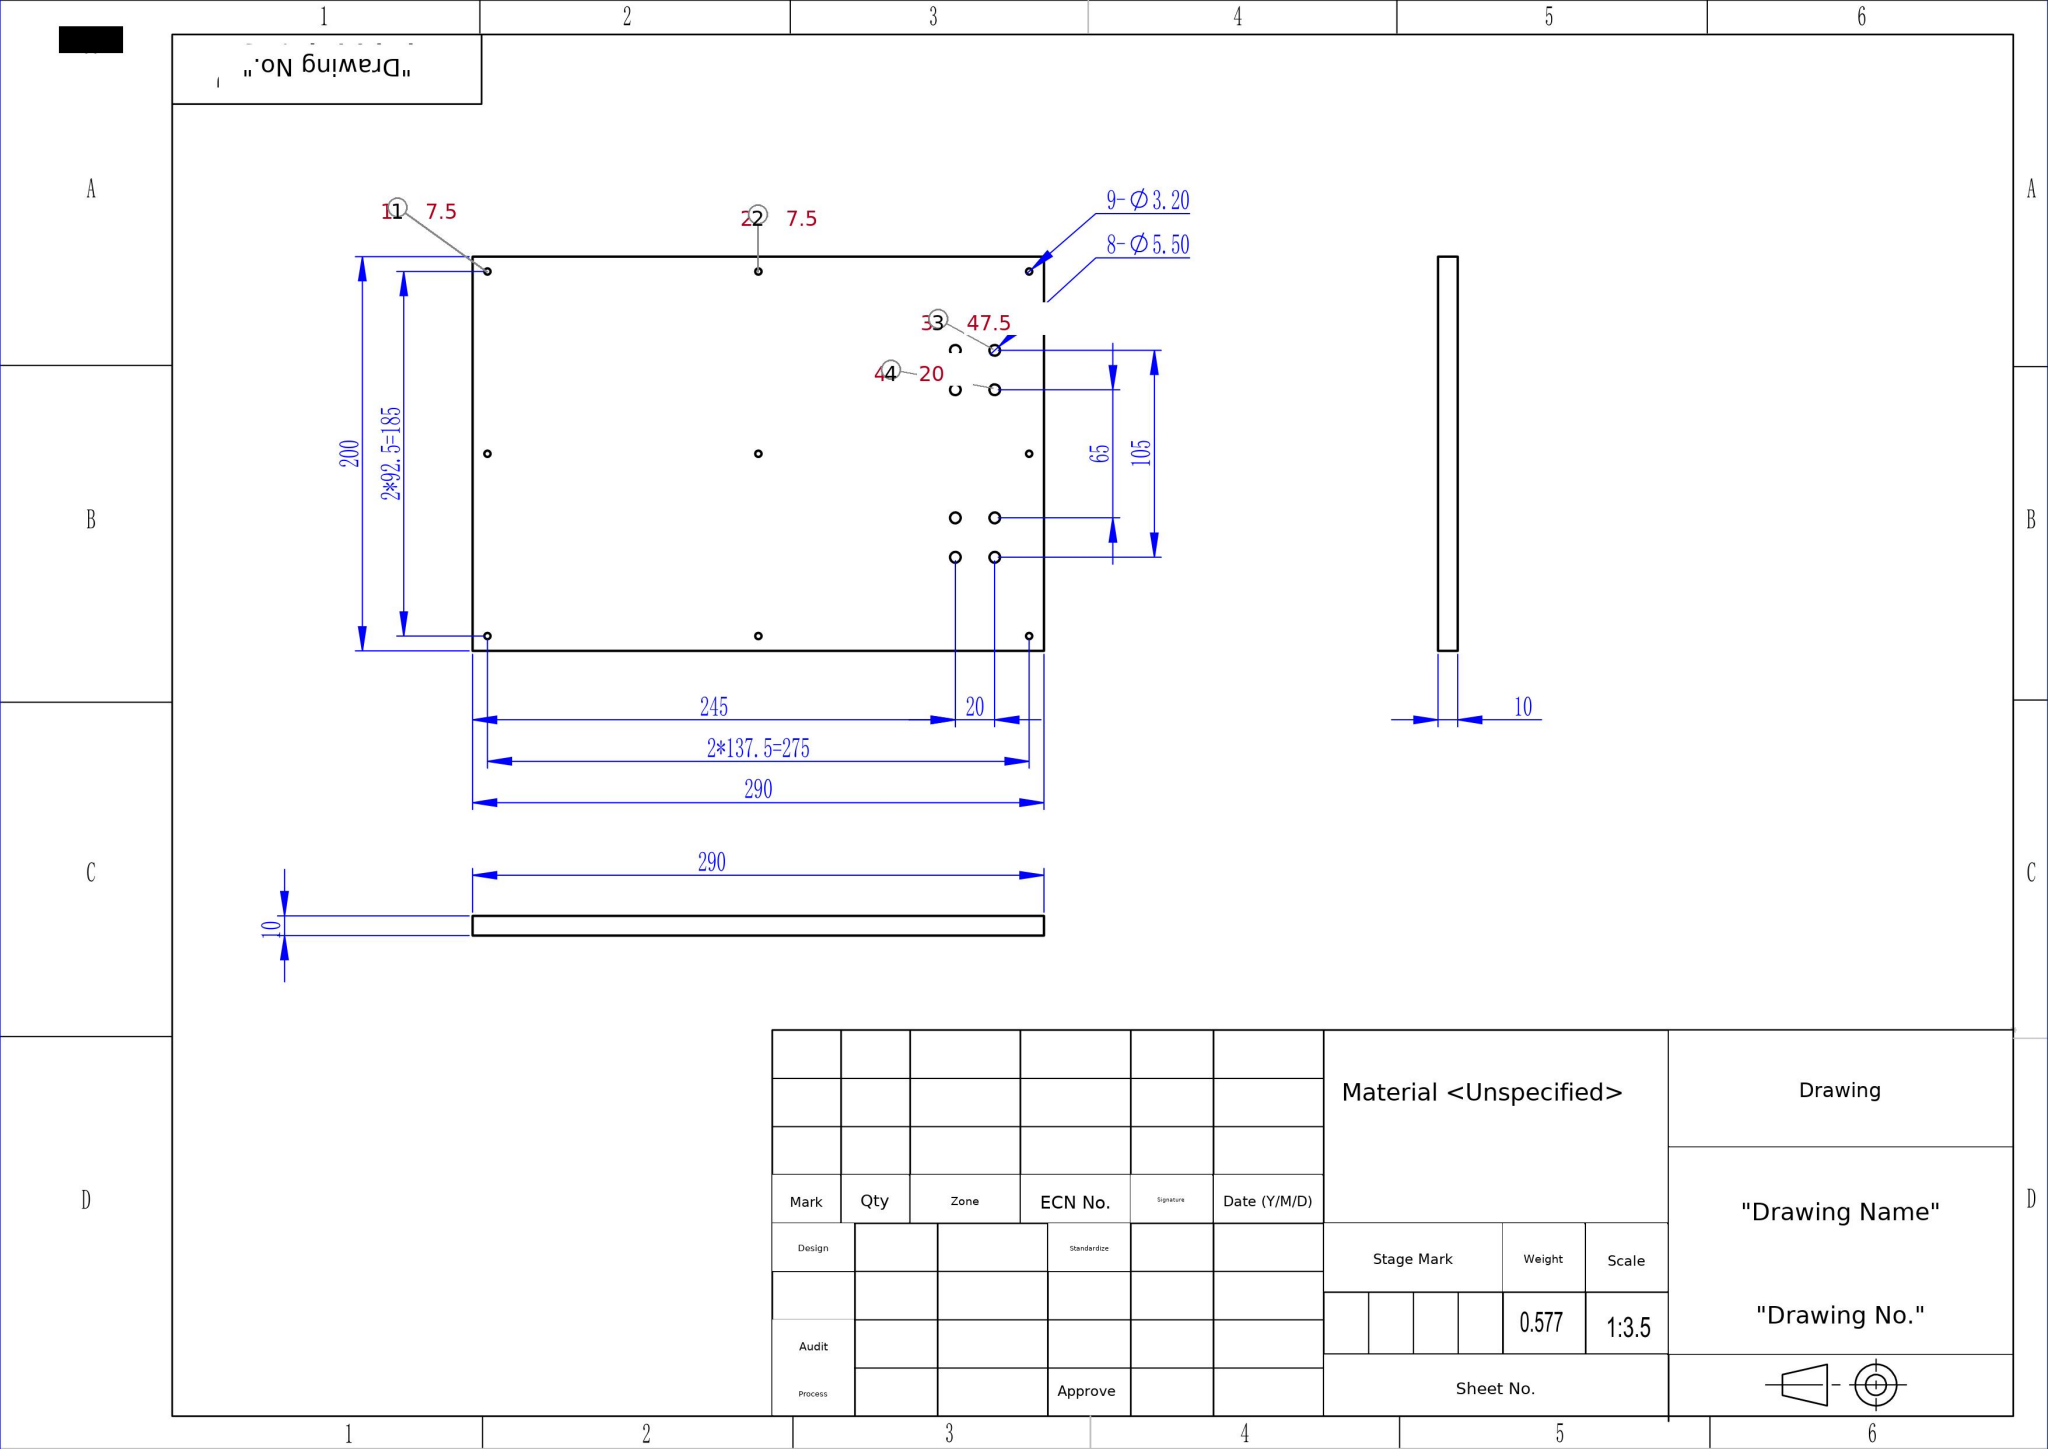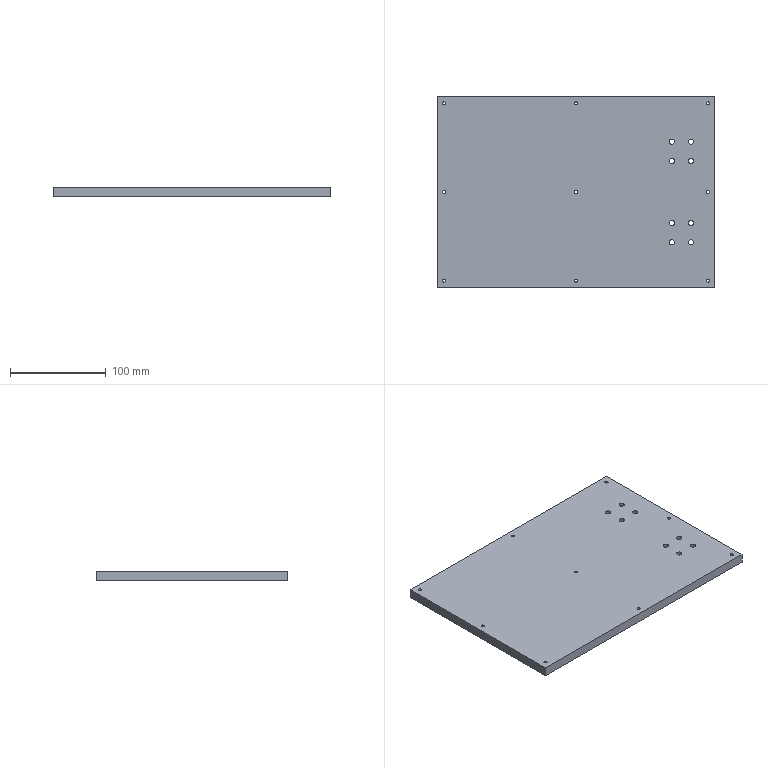Part | SolidWorks | mm | material Unspecified | 1 solid | 40 faces | box 290 x 200 x 10 mm | volume 577376 mm3 | cylinder 34 | plane 6 | commonest cylinder face diameters 3.2 x18 5.5 x16
build123d program:
from build123d import *

# Parameters (mm, degrees)
MODEL_W             = 290
MODEL_H             = 200
MODEL_R             = 2.75
MODEL_R_2           = 1.6
BOSS_EXTRUDE1_DEPTH = 10


with BuildPart() as part:
    # Model → Boss-Extrude1 (new body)
    with BuildSketch(Plane.XY):
        with Locations((642.697, 272.461)):
            Rectangle(MODEL_W, MODEL_H)
        with Locations((742.697, 219.961)):
            Circle(MODEL_R, mode=Mode.SUBTRACT)
        with Locations((762.697, 219.961)):
            Circle(MODEL_R, mode=Mode.SUBTRACT)
        with Locations((742.697, 239.961)):
            Circle(MODEL_R, mode=Mode.SUBTRACT)
        with Locations((762.697, 239.961)):
            Circle(MODEL_R, mode=Mode.SUBTRACT)
        with Locations((742.697, 324.961)):
            Circle(MODEL_R, mode=Mode.SUBTRACT)
        with Locations((762.697, 324.961)):
            Circle(MODEL_R, mode=Mode.SUBTRACT)
        with Locations((742.697, 304.961)):
            Circle(MODEL_R, mode=Mode.SUBTRACT)
        with Locations((762.697, 304.961)):
            Circle(MODEL_R, mode=Mode.SUBTRACT)
        with Locations((642.697, 364.961)):
            Circle(MODEL_R_2, mode=Mode.SUBTRACT)
        with Locations((642.697, 179.961)):
            Circle(MODEL_R_2, mode=Mode.SUBTRACT)
        with Locations((505.197, 272.461)):
            Circle(MODEL_R_2, mode=Mode.SUBTRACT)
        with Locations((780.197, 272.461)):
            Circle(MODEL_R_2, mode=Mode.SUBTRACT)
        with Locations((642.697, 272.461)):
            Circle(MODEL_R_2, mode=Mode.SUBTRACT)
        with Locations((780.197, 364.961)):
            Circle(MODEL_R_2, mode=Mode.SUBTRACT)
        with Locations((505.197, 364.961)):
            Circle(MODEL_R_2, mode=Mode.SUBTRACT)
        with Locations((780.197, 179.961)):
            Circle(MODEL_R_2, mode=Mode.SUBTRACT)
        with Locations((505.197, 179.961)):
            Circle(MODEL_R_2, mode=Mode.SUBTRACT)
    extrude(amount=BOSS_EXTRUDE1_DEPTH)


solid = part.part